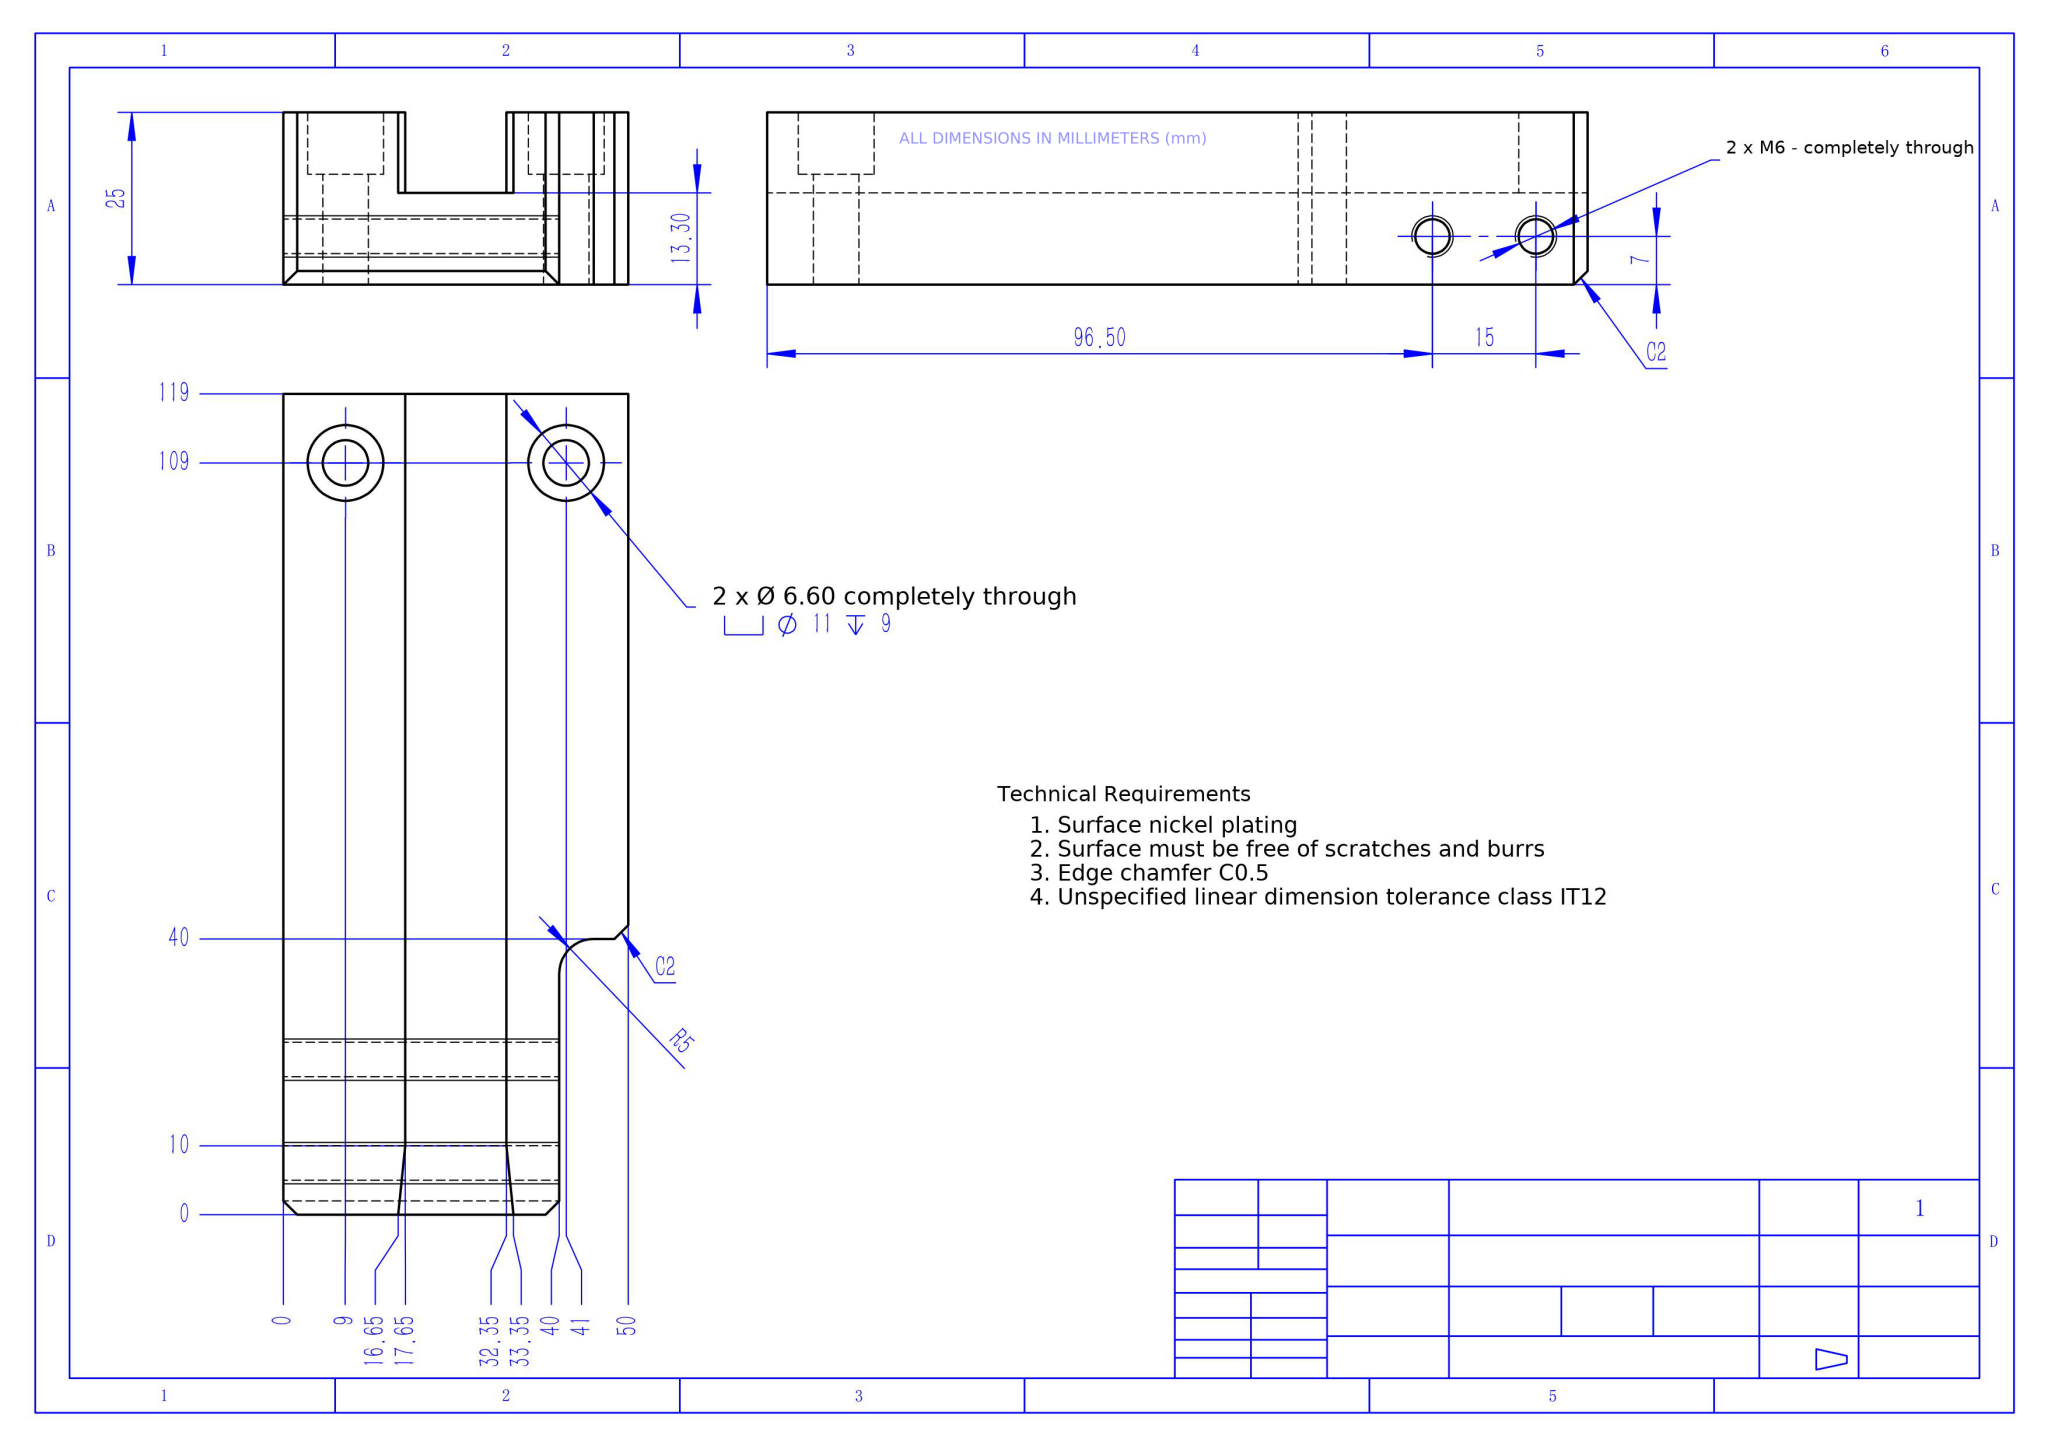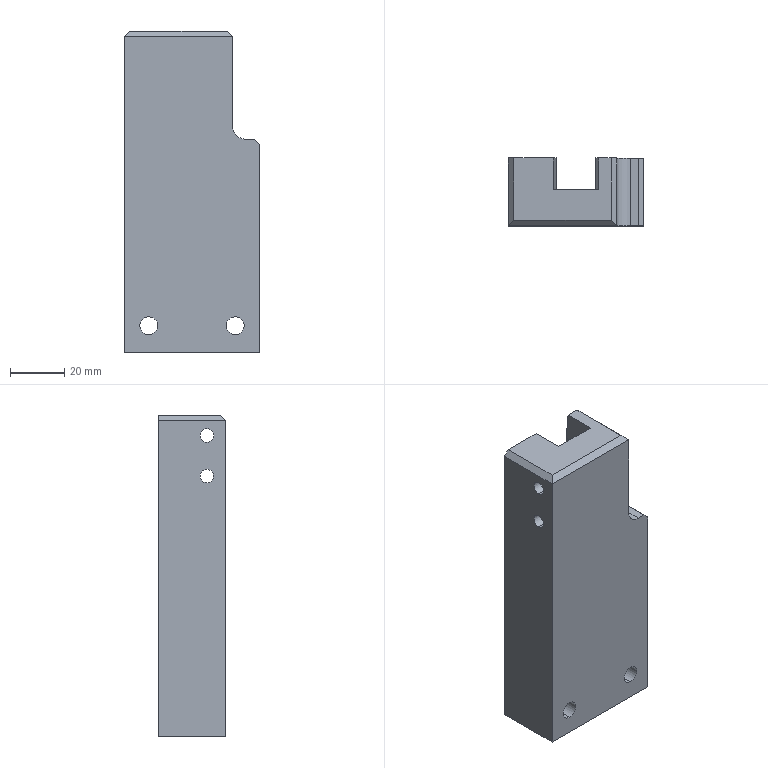Part | NX | mm | 1 solid | 33 faces | box 50 x 25 x 119 mm | volume 113699 mm3 | plane 20 | cylinder 13 | commonest cylinder face diameters 5 x4 11 x4 6.6 x4 10 x1